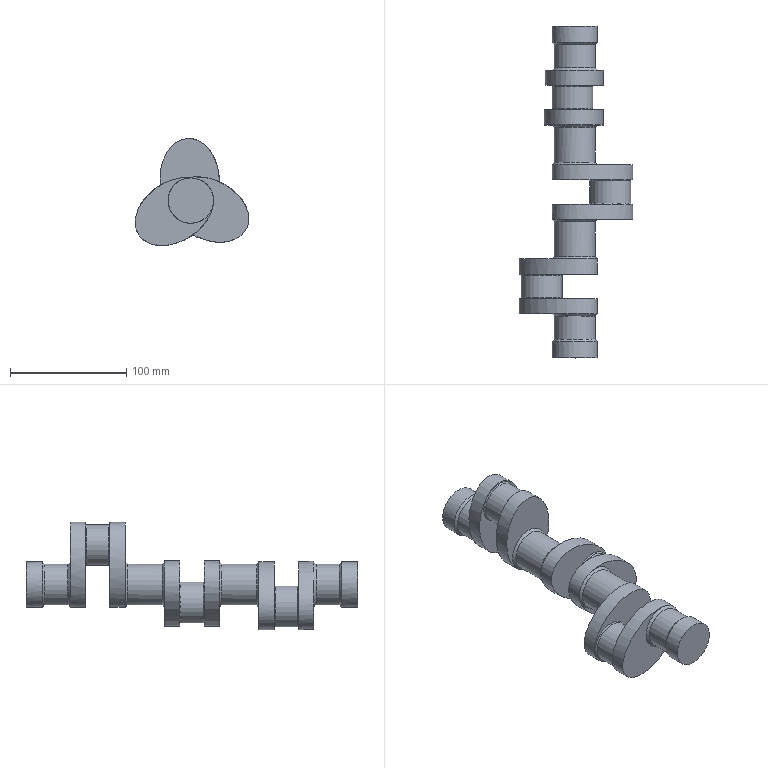Component | NX | CRANKSHAFT | 1 solid | 45 faces | volume 435321 mm3 | plane 16 | cone 14 | cylinder 9 | other 6 | commonest cylinder face diameters 35 x7 39 x2